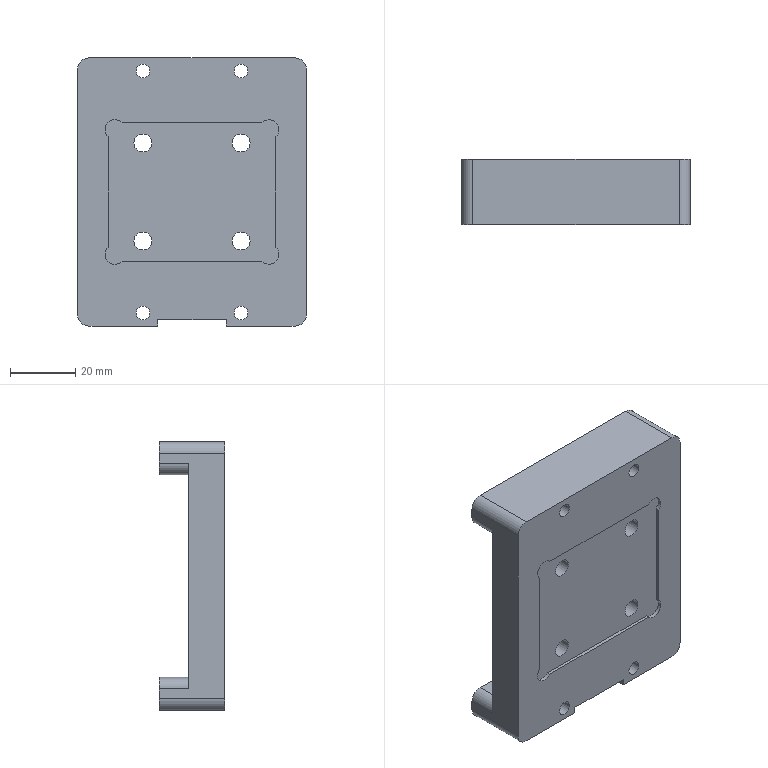Component | SolidWorks | KKConnectingPlate-3-1 | 1 solid | 69 faces | box 70 x 20 x 82 mm | volume 69082 mm3 | cylinder 42 | plane 23 | cone 4 | commonest cylinder face diameters 10 x8 4.2 x8 5.5 x8 7 x8 6 x6 3.3 x4
build123d program:
from build123d import *

# Parameters (mm, degrees)
SKETCH1_W                                       = 70
SKETCH1_H                                       = 82
BOSS_EXTRUDE1_DEPTH                             = 10
SKETCH2_W                                       = 70
SKETCH2_H                                       = 10
BOSS_EXTRUDE2_DEPTH                             = 9
M5_TAPPED_HOLE1_D                               = 4.2
M5_HEX_SOCKET_HEAD_CAP_SCREW_CBORE1_D           = 5.5
M5_HEX_SOCKET_HEAD_CAP_SCREW_CBORE1_CBORE_D     = 10
M5_HEX_SOCKET_HEAD_CAP_SCREW_CBORE1_CBORE_DEPTH = 5
BOSS_EXTRUDE3_START                             = 1
SKETCH7_W                                       = 70
SKETCH7_H                                       = 82
SKETCH7_R                                       = 2.1
SKETCH7_R_2                                     = 2.75
BOSS_EXTRUDE3_DEPTH                             = 1
SKETCH8_W                                       = 51.2
SKETCH8_H                                       = 42.2
CUT_EXTRUDE1_DEPTH                              = 1
SKETCH9_R                                       = 3
CUT_EXTRUDE2_DEPTH                              = 1
SKETCH10_W                                      = 21
SKETCH10_H                                      = 28.111
CUT_EXTRUDE3_DEPTH                              = 2
M4_TAPPED_HOLE1_D                               = 3.3
M4_TAPPED_HOLE1_DEPTH                           = 10.1
M4_TAPPED_HOLE1_TIP                             = 0.9914
FILLET2_R                                       = 3.5


with BuildPart() as part:
    # Sketch1 → Boss-Extrude1 (new body)
    with BuildSketch(Plane.XY):
        with Locations((-79, 0)):
            Rectangle(SKETCH1_W, SKETCH1_H)
    extrude(amount=BOSS_EXTRUDE1_DEPTH)

    # Sketch2 → Boss-Extrude2 (add)
    with BuildSketch(Plane.XY.offset(10)):
        with Locations((-79, 36)):
            Rectangle(SKETCH2_W, SKETCH2_H)
        with Locations((-79, -36)):
            Rectangle(SKETCH2_W, SKETCH2_H)
    extrude(amount=BOSS_EXTRUDE2_DEPTH)

    # M5 Tapped Hole1 (through all)
    with Locations(Plane.XY.offset(19)):
        with Locations((-94, 37), (-64, 37), (-94, -37), (-64, -37)):
            Hole(M5_TAPPED_HOLE1_D / 2)

    # M5 Hex Socket Head Cap Screw CBORE1 (through all)
    with Locations(Plane.XY.offset(10)):
        with Locations((-94, 15), (-64, 15), (-64, -15), (-94, -15)):
            CounterBoreHole(M5_HEX_SOCKET_HEAD_CAP_SCREW_CBORE1_D / 2, M5_HEX_SOCKET_HEAD_CAP_SCREW_CBORE1_CBORE_D / 2, M5_HEX_SOCKET_HEAD_CAP_SCREW_CBORE1_CBORE_DEPTH)

    # Sketch7 → Boss-Extrude3 (add)
    with BuildSketch(Plane(origin=(0, 0, 0), x_dir=(-1, 0, 0), z_dir=(0, 0, -1)).offset(BOSS_EXTRUDE3_START)):
        with Locations((79, 0)):
            Rectangle(SKETCH7_W, SKETCH7_H)
        with Locations(Location((94, 37, 0), (0, 0, 180))):
            Circle(SKETCH7_R, mode=Mode.SUBTRACT)
        with Locations(Location((64, 37, 0), (0, 0, 180))):
            Circle(SKETCH7_R, mode=Mode.SUBTRACT)
        with Locations(Location((94, 15, 0), (0, 0, 180))):
            Circle(SKETCH7_R_2, mode=Mode.SUBTRACT)
        with Locations(Location((64, 15, 0), (0, 0, 180))):
            Circle(SKETCH7_R_2, mode=Mode.SUBTRACT)
        with Locations(Location((64, -15, 0), (0, 0, 180))):
            Circle(SKETCH7_R_2, mode=Mode.SUBTRACT)
        with Locations(Location((94, -15, 0), (0, 0, 180))):
            Circle(SKETCH7_R_2, mode=Mode.SUBTRACT)
        with Locations(Location((94, -37, 0), (0, 0, 180))):
            Circle(SKETCH7_R, mode=Mode.SUBTRACT)
        with Locations(Location((64, -37, 0), (0, 0, 180))):
            Circle(SKETCH7_R, mode=Mode.SUBTRACT)
    extrude(amount=-BOSS_EXTRUDE3_DEPTH)

    # Sketch8 → Cut-Extrude1 (cut)
    with BuildSketch(Plane(origin=(0, 0, -1), x_dir=(-1, 0, 0), z_dir=(0, 0, -1))):
        with Locations((79, 0)):
            Rectangle(SKETCH8_W, SKETCH8_H)
    extrude(amount=-CUT_EXTRUDE1_DEPTH, mode=Mode.SUBTRACT)

    # Sketch9 → Cut-Extrude2 (cut)
    with BuildSketch(Plane(origin=(0, 0, 0), x_dir=(-1, 0, 0), z_dir=(0, 0, -1))):
        with Locations((55.4, 19.1)):
            Circle(SKETCH9_R)
        with Locations((102.6, 19.1)):
            Circle(SKETCH9_R)
        with Locations((55.4, -19.1)):
            Circle(SKETCH9_R)
        with Locations((102.6, -19.1)):
            Circle(SKETCH9_R)
    extrude(amount=CUT_EXTRUDE2_DEPTH, mode=Mode.SUBTRACT)

    # Sketch10 → Cut-Extrude3 (cut)
    with BuildSketch(Plane(origin=(0, 41, 0), x_dir=(1, 0, 0), z_dir=(0, 1, 0))):
        with Locations((-79, -9)):
            Rectangle(SKETCH10_W, SKETCH10_H)
    extrude(amount=-CUT_EXTRUDE3_DEPTH, mode=Mode.SUBTRACT)

    # M4 Tapped Hole1
    with Locations(Plane(origin=(0, 39, 0), x_dir=(1, 0, 0), z_dir=(0, 1, 0))):
        with Locations((-84, -9), (-74, -9)):
            Hole(M4_TAPPED_HOLE1_D / 2, depth=M4_TAPPED_HOLE1_DEPTH)
            with Locations((0, 0, -(M4_TAPPED_HOLE1_DEPTH + M4_TAPPED_HOLE1_TIP / 2))):  # 118° drill point
                Cone(0, M4_TAPPED_HOLE1_D / 2, M4_TAPPED_HOLE1_TIP, mode=Mode.SUBTRACT)

    # Fillet2
    fillet2_edges = [part.edges().sort_by_distance(p)[0] for p in [
        (-114, 31, 14.5),
        (-44, 31, 14.5),
        (-114, -31, 14.5),
        (-44, -31, 14.5),
        (-44, -41, 9),
        (-114, -41, 9),
        (-114, 41, 9),
        (-44, 41, 9),
    ]]
    fillet(fillet2_edges, radius=FILLET2_R)


solid = part.part

# Placed as in the assembly
solid = solid.moved(Location((55.019, 23.016, 82), (-90, 0, 0)))